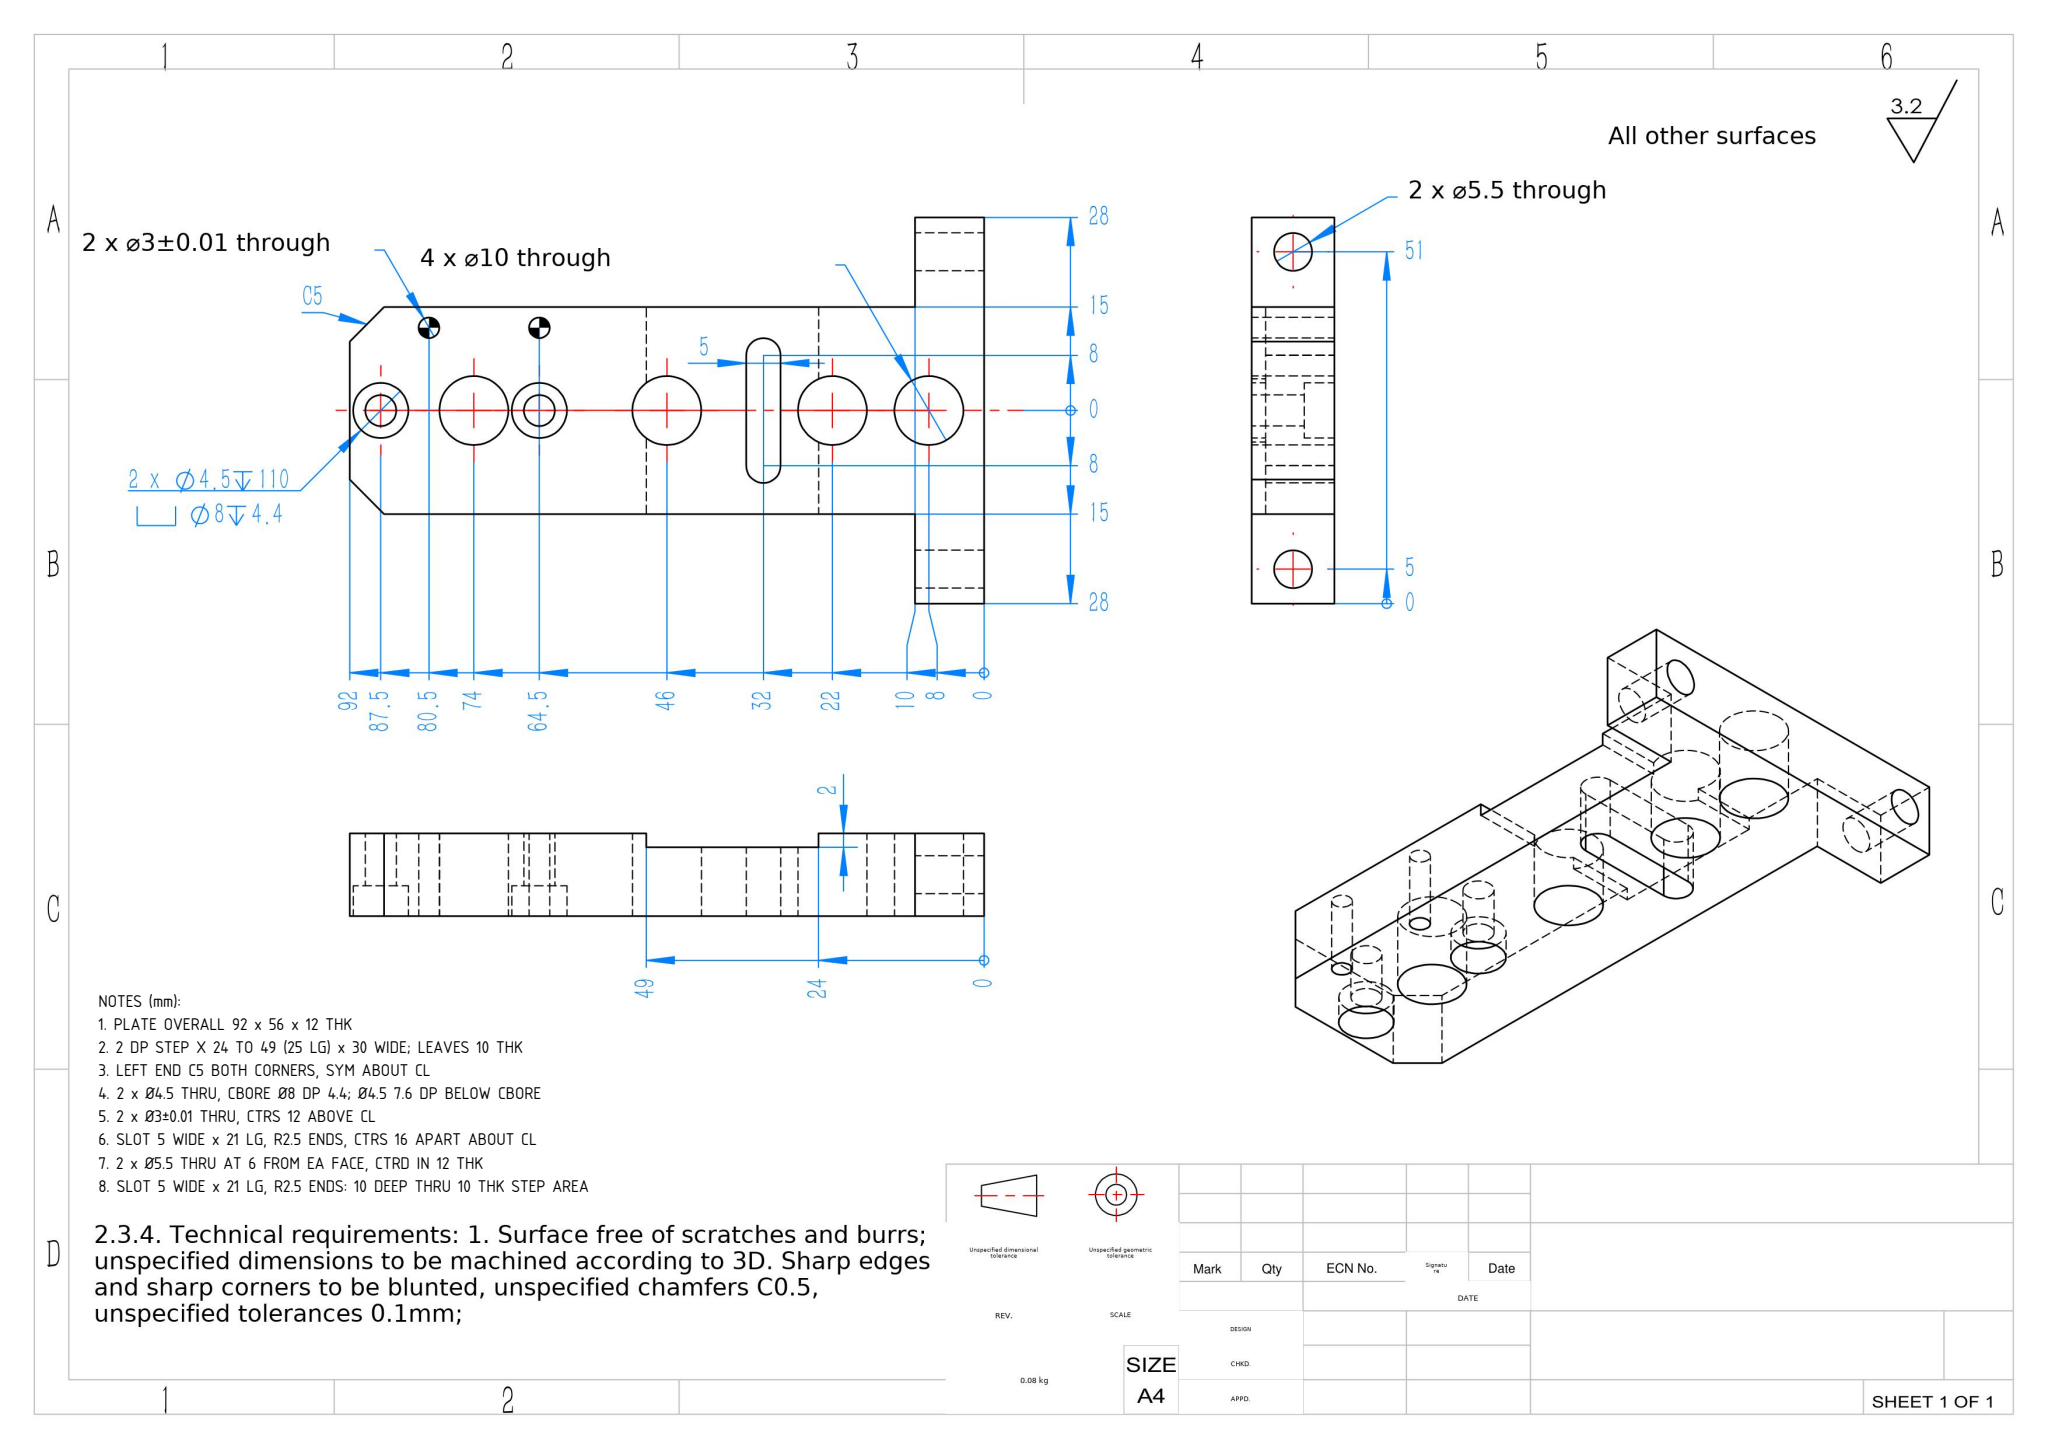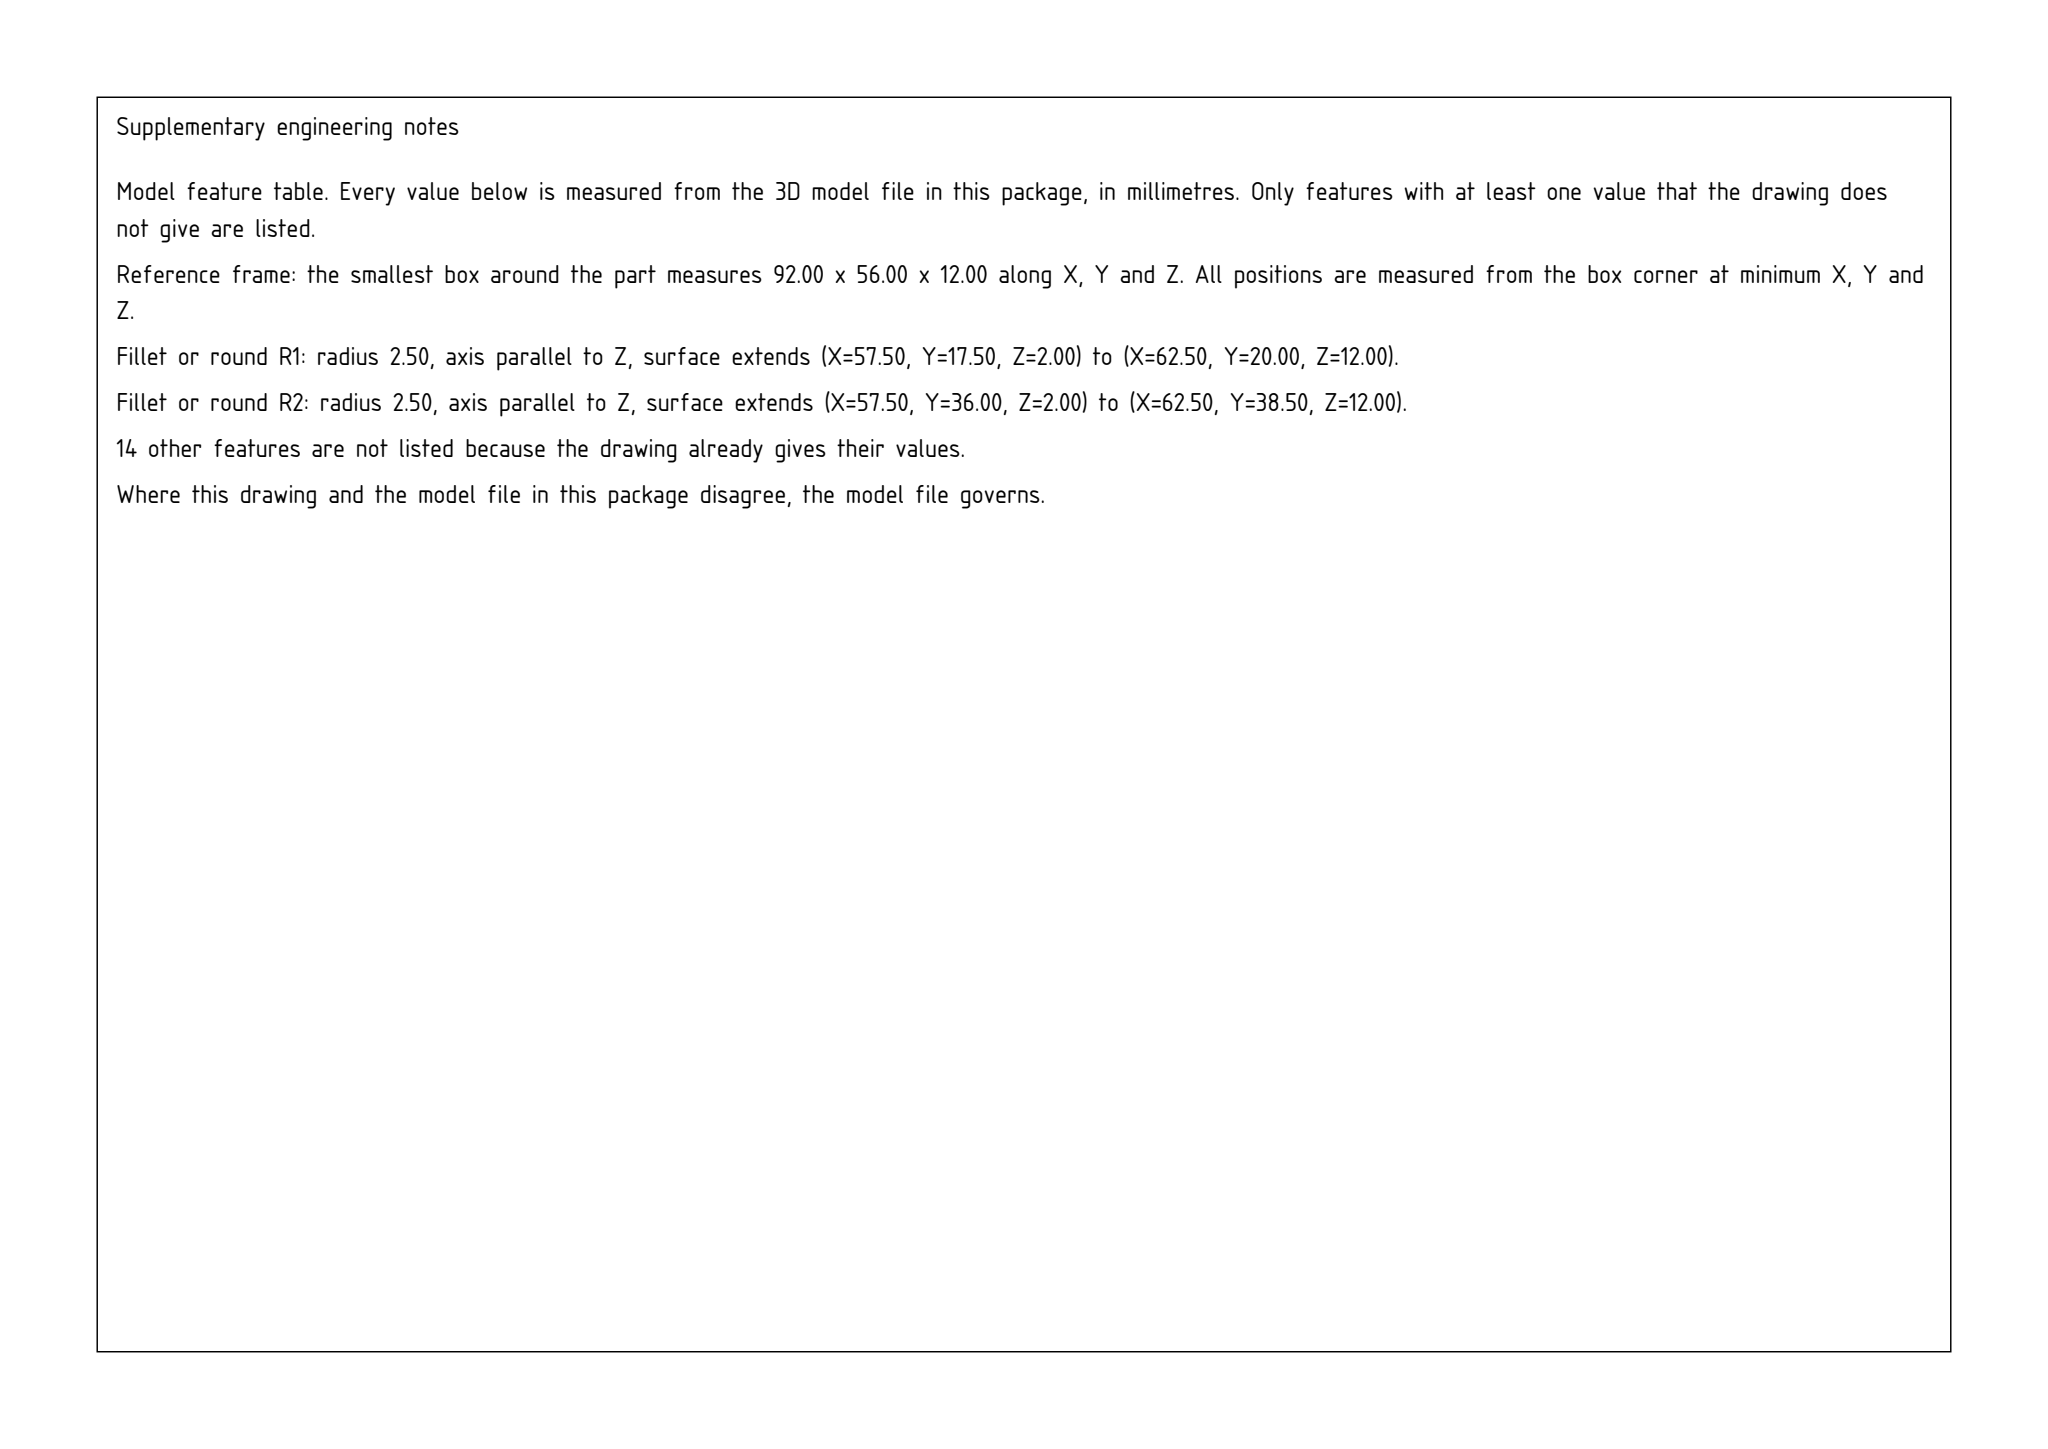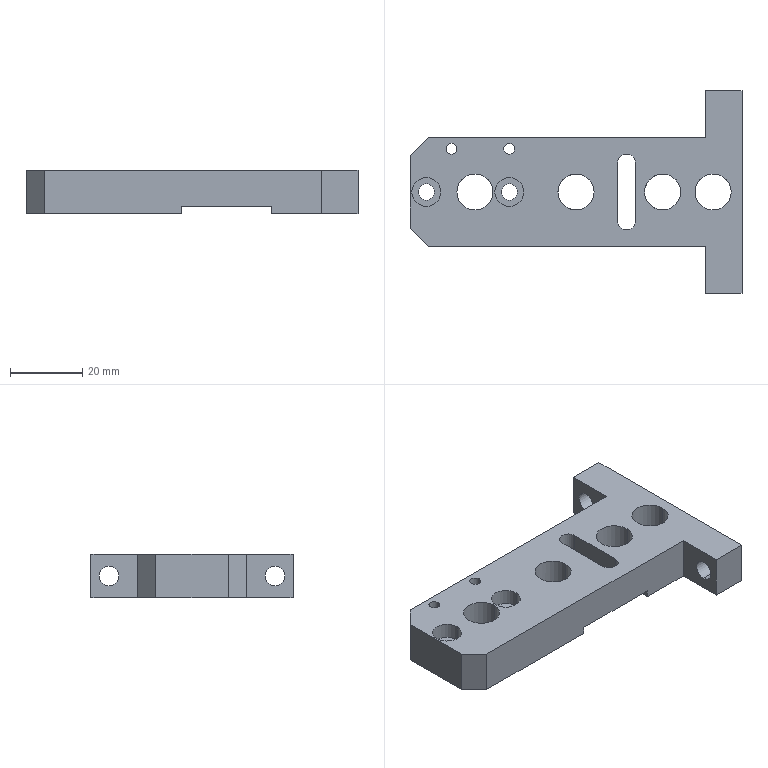Part | SolidWorks | mm | 1 solid | 48 faces | box 92 x 56 x 12 mm | volume 28519 mm3 | cylinder 26 | plane 22 | commonest cylinder face diameters 10 x8 3 x4 8 x4 4.5 x4 5.5 x4 5 x2
Drawing notes:
PLATE OVERALL 92 x 56 x 12 THK | from the solid: bbox_xyz [92.0,56.0,12.0]
2 DP STEP X 24 TO 49 (25 LG) x 30 WIDE; LEAVES 10 THK | from the solid: x planes 43 & 68 (24/49 from right datum), y 13-43, z faces 0/2/12
LEFT END C5 BOTH CORNERS, SYM ABOUT CL | from the solid: y planes 13 & 43 sym about hole CL y=28; end face x=0
2 x Ø4.5 THRU, CBORE Ø8 DP 4.4; Ø4.5 7.6 DP BELOW CBORE | from the solid: Ø4.5 z-cyl len 7.6 + Ø8 z-cyl len 4.4 = 12 plate thk; cbore floor z=7.6
2 x Ø3±0.01 THRU, CTRS 12 ABOVE CL | from the solid: Ø3 z-cyls at y=40.0; part CL y=28.0 (56 wide)
SLOT 5 WIDE x 21 LG, R2.5 ENDS, CTRS 16 APART ABOUT CL | from the solid: Ø5 z-cyls at (60,20) & (60,36); x planes 57.5 & 62.5; CL y=28
2 x Ø5.5 THRU AT 6 FROM EA FACE, CTRD IN 12 THK | from the solid: Ø5.5 x-axis cyls at z=6, plate z 0-12
SLOT 5 WIDE x 21 LG, R2.5 ENDS: 10 DEEP THRU 10 THK STEP AREA | from the solid: Two Ø5 z-axis cylinders at (60,20) & (60,36), length 10, in 2 mm step region (z plane 2.0 to 12.0) = slot 5 wide, 21 end-to-end, breaking through 10 mm remaining thickness
build123d program:
from build123d import *

# Parameters (mm, degrees)
SKETCH1_W                                       = 92
SKETCH1_H                                       = 56
BOSS_EXTRUDE1_DEPTH                             = 6
SKETCH2_W                                       = 82
SKETCH2_H                                       = 13
CUT_EXTRUDE1_DEPTH                              = 56.172
F_5_5_5_5_DIAMETER_HOLE1_D                      = 5.5
M4_HEX_SOCKET_HEAD_CAP_SCREW_CBORE1_D           = 4.5
M4_HEX_SOCKET_HEAD_CAP_SCREW_CBORE1_DEPTH       = 110
M4_HEX_SOCKET_HEAD_CAP_SCREW_CBORE1_CBORE_D     = 8
M4_HEX_SOCKET_HEAD_CAP_SCREW_CBORE1_CBORE_DEPTH = 4.4
M4_HEX_SOCKET_HEAD_CAP_SCREW_CBORE1_TIP         = 1.352
CUT_EXTRUDE2_DEPTH                              = 56.172
SIZE_MM_DOWEL_PIN_HOLE_1_D                      = 3
F_10_0_10_DIAMETER_HOLE1_D                      = 10
CHAMFER1_SIZE                                   = 5
SKETCH19_W                                      = 25
SKETCH19_H                                      = 2
CUT_EXTRUDE3_DEPTH                              = 64.253


with BuildPart() as part:
    # Sketch1 → Boss-Extrude1 (new, symmetric)
    with BuildSketch(Plane.XY):
        Rectangle(SKETCH1_W, SKETCH1_H)
    extrude(amount=BOSS_EXTRUDE1_DEPTH, both=True)

    # Sketch2 → Cut-Extrude1 (cut, through all)
    with BuildSketch(Plane.XY.offset(6)):
        with Locations((-5, 21.5)):
            Rectangle(SKETCH2_W, SKETCH2_H)
        with Locations((-5, -21.5)):
            Rectangle(SKETCH2_W, SKETCH2_H)
    extrude(amount=-CUT_EXTRUDE1_DEPTH, mode=Mode.SUBTRACT)

    # 5.5 _5.5_ Diameter Hole1 (through all)
    with Locations(Plane.ZY.offset(-36)):
        with Locations((0, -23), (0, 23)):
            Hole(F_5_5_5_5_DIAMETER_HOLE1_D / 2)

    # M4 Hex Socket Head Cap Screw CBORE1
    with Locations(Plane.XY.offset(6)):
        with Locations((-41.5, 0), (-18.5, 0)):
            CounterBoreHole(M4_HEX_SOCKET_HEAD_CAP_SCREW_CBORE1_D / 2, M4_HEX_SOCKET_HEAD_CAP_SCREW_CBORE1_CBORE_D / 2, M4_HEX_SOCKET_HEAD_CAP_SCREW_CBORE1_CBORE_DEPTH, depth=M4_HEX_SOCKET_HEAD_CAP_SCREW_CBORE1_DEPTH)
            with Locations((0, 0, -(M4_HEX_SOCKET_HEAD_CAP_SCREW_CBORE1_DEPTH + M4_HEX_SOCKET_HEAD_CAP_SCREW_CBORE1_TIP / 2))):  # 118° drill point
                Cone(0, M4_HEX_SOCKET_HEAD_CAP_SCREW_CBORE1_D / 2, M4_HEX_SOCKET_HEAD_CAP_SCREW_CBORE1_TIP, mode=Mode.SUBTRACT)

    # Sketch9 → Cut-Extrude2 (cut, through all)
    with BuildSketch(Plane.XY.offset(6)):
        with BuildLine():
            Line((11.5, -8), (11.5, 8))
            ThreePointArc((11.5, 8), (14, 10.5), (16.5, 8))
            Line((16.5, 8), (16.5, -8))
            ThreePointArc((16.5, -8), (14, -10.5), (11.5, -8))
        make_face()
    extrude(amount=-CUT_EXTRUDE2_DEPTH, mode=Mode.SUBTRACT)

    # Size mm Dowel Pin Hole 1 (through all)
    with Locations(Plane.XY.offset(6)):
        with Locations((-34.5, 12), (-18.5, 12)):
            Hole(SIZE_MM_DOWEL_PIN_HOLE_1_D / 2)

    # 10.0 _10_ Diameter Hole1 (through all)
    with Locations(Plane.XY.offset(6)):
        with Locations((-28, 0), (38, 0), (0, 0), (24, 0)):
            Hole(F_10_0_10_DIAMETER_HOLE1_D / 2)

    # Chamfer1
    chamfer1_edges = [part.edges().sort_by_distance(p)[0] for p in [
        (-46, 15, 0),
        (-46, -15, 0),
    ]]
    chamfer(chamfer1_edges, length=CHAMFER1_SIZE)

    # Sketch19 → Cut-Extrude3 (cut, through all)
    with BuildSketch(Plane(origin=(0, 15, 0), x_dir=(1, 0, 0), z_dir=(0, 1, 0))):
        with Locations((9.5, 5)):
            Rectangle(SKETCH19_W, SKETCH19_H)
    extrude(amount=-CUT_EXTRUDE3_DEPTH, mode=Mode.SUBTRACT)


solid = part.part